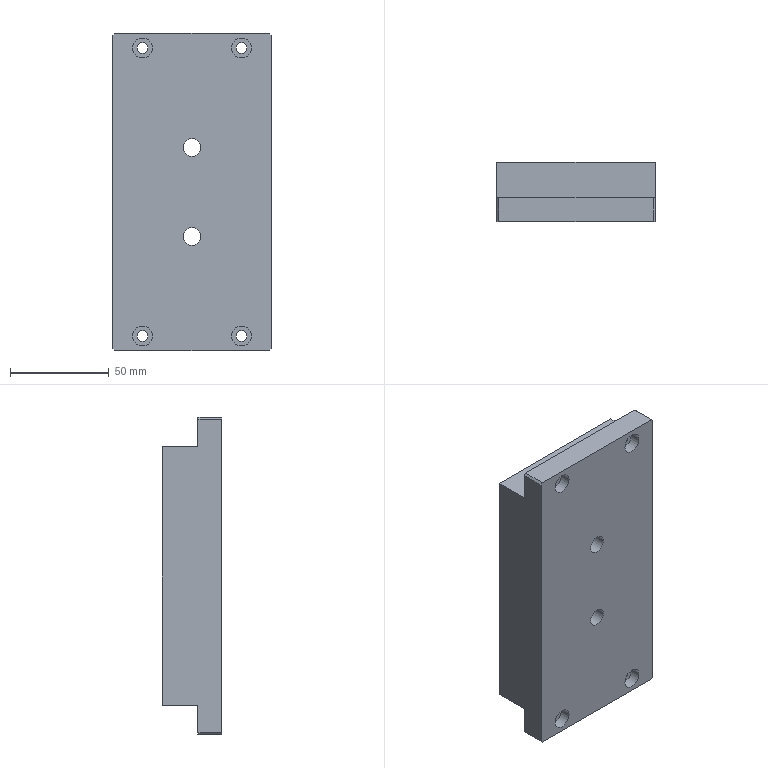Component | SolidWorks | XT-1-03-2-1 | 1 solid | 44 faces | box 80 x 30 x 160.5 mm | volume 332442 mm3 | cylinder 24 | plane 20 | commonest cylinder face diameters 10 x8 5.5 x8 15 x4 9 x4
build123d program:
from build123d import *

# Parameters (mm, degrees)
BOSS_EXTRUDE1_DEPTH                             = 80
M5_HEX_SOCKET_HEAD_CAP_SCREW_CBORE1_D           = 5.5
M5_HEX_SOCKET_HEAD_CAP_SCREW_CBORE1_CBORE_D     = 10
M5_HEX_SOCKET_HEAD_CAP_SCREW_CBORE1_CBORE_DEPTH = 5.4
M8_HEX_SOCKET_HEAD_CAP_SCREW_CBORE1_D           = 9
M8_HEX_SOCKET_HEAD_CAP_SCREW_CBORE1_CBORE_D     = 15
M8_HEX_SOCKET_HEAD_CAP_SCREW_CBORE1_CBORE_DEPTH = 15
CHAMFER1_SIZE                                   = 1


with BuildPart() as part:
    # Sketch1 → Boss-Extrude1 (new body)
    with BuildSketch(Plane.XY):
        Polygon((0, 0), (0, -12), (160.5, -12), (160.5, 0), (145.5, 0), (145.5, 18), (15, 18), (15, 0), align=None)
    extrude(amount=BOSS_EXTRUDE1_DEPTH)

    # M5 Hex Socket Head Cap Screw CBORE1 (through all)
    with Locations(Plane(origin=(0, -12, 0), x_dir=(-1, 0, 0), z_dir=(0, -1, 0))):
        with Locations((-7.5, -15), (-7.5, -65), (-153, -15), (-153, -65)):
            CounterBoreHole(M5_HEX_SOCKET_HEAD_CAP_SCREW_CBORE1_D / 2, M5_HEX_SOCKET_HEAD_CAP_SCREW_CBORE1_CBORE_D / 2, M5_HEX_SOCKET_HEAD_CAP_SCREW_CBORE1_CBORE_DEPTH)

    # M8 Hex Socket Head Cap Screw CBORE1 (through all)
    with Locations(Plane(origin=(0, 18, 0), x_dir=(1, 0, 0), z_dir=(0, 1, 0))):
        with Locations((57.75, -40), (102.75, -40)):
            CounterBoreHole(M8_HEX_SOCKET_HEAD_CAP_SCREW_CBORE1_D / 2, M8_HEX_SOCKET_HEAD_CAP_SCREW_CBORE1_CBORE_D / 2, M8_HEX_SOCKET_HEAD_CAP_SCREW_CBORE1_CBORE_DEPTH)

    # Chamfer1
    chamfer1_edges = [part.edges().sort_by_distance(p)[0] for p in [
        (0, -6, 0),
        (160.5, -6, 80),
        (0, -6, 80),
        (160.5, -6, 0),
    ]]
    chamfer(chamfer1_edges, length=CHAMFER1_SIZE)


solid = part.part

# Placed as in the assembly
solid = solid.moved(Location((254.283, 54.385, 7.5), (0, 90, 0)))